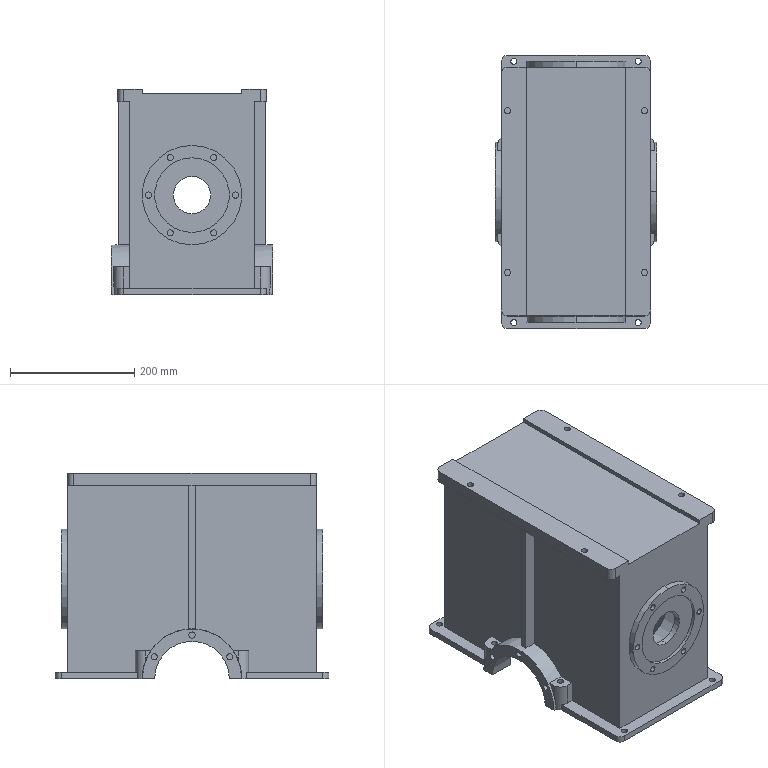Component | SolidWorks | WormGearReducerLowerCasing-1 | 1 solid | 189 faces | volume 6052719 mm3 | cylinder 105 | plane 80 | cone 4 | commonest cylinder face diameters 10 x60 160 x11 120 x10 15 x8 20 x8 60 x4 32 x4